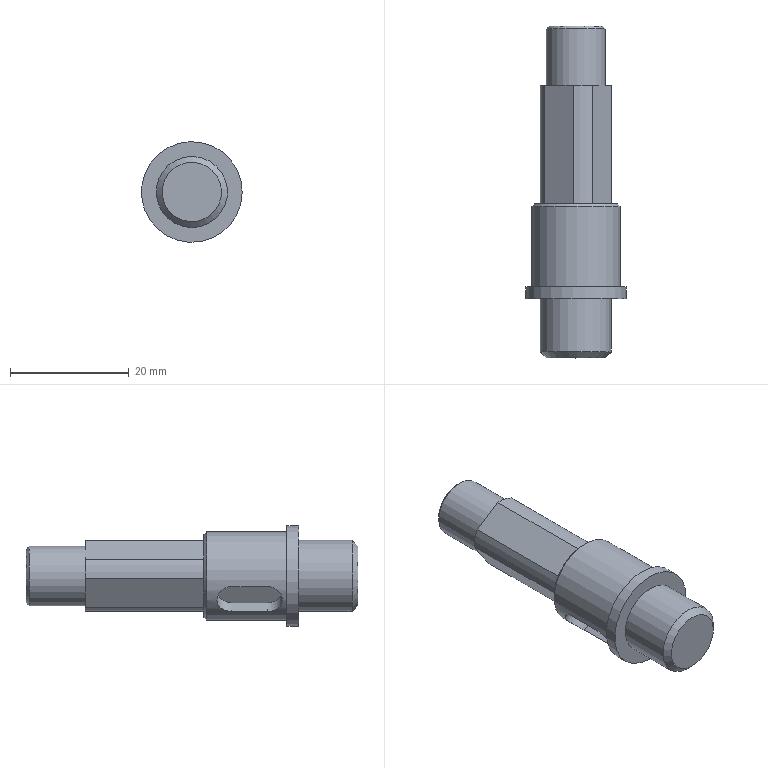Component | NX | CLHKJG_05_INPUT_SHAFT | 1 solid | 26 faces | volume 6700 mm3 | plane 13 | cylinder 10 | cone 3 | commonest cylinder face diameters 12 x5 5 x2 17 x1 15 x1 10 x1